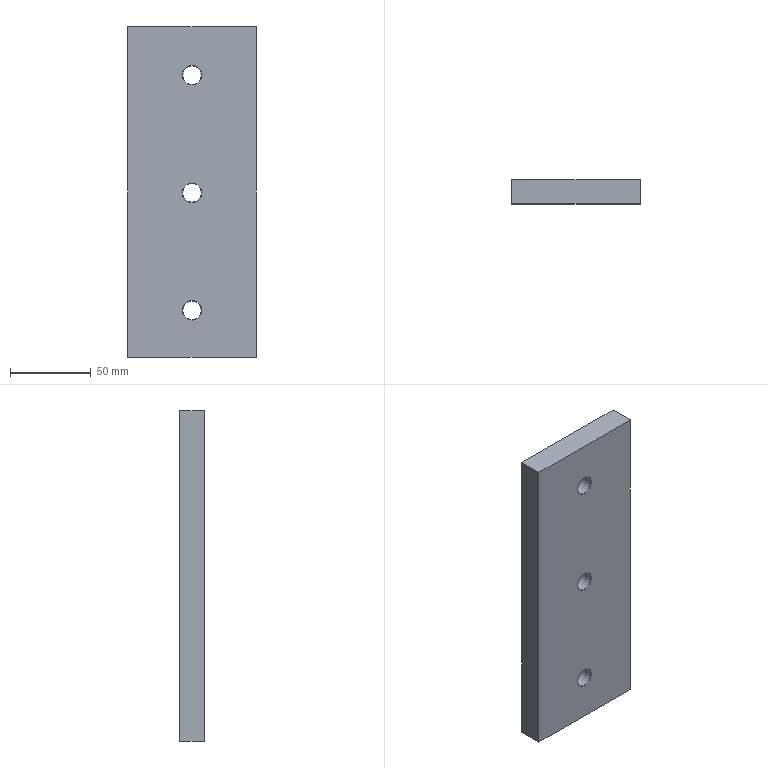Component | NX | CH3404_5-13_2 | 1 solid | 15 faces | box 80 x 15 x 205 mm | volume 241319 mm3 | plane 6 | cone 6 | cylinder 3 | commonest cylinder face diameters 11.5 x3
STEP:
#1=CARTESIAN_POINT('',(0.,0.,0.));
#2=DIRECTION('',(0.,0.,1.));
#3=DIRECTION('',(1.,0.,0.));
#4=AXIS2_PLACEMENT_3D('',#1,#2,#3);
#5=CARTESIAN_POINT('',(-275.,172.5,-10.));
#6=VERTEX_POINT('',#5);
#7=CARTESIAN_POINT('',(-275.,172.5,-215.));
#8=VERTEX_POINT('',#7);
#9=CARTESIAN_POINT('',(-275.,172.5,-10.));
#10=DIRECTION('',(0.,0.,-1.));
#11=VECTOR('',#10,1.);
#12=LINE('',#9,#11);
#13=CARTESIAN_POINT('',(-275.,187.5,-10.));
#14=DIRECTION('',(-1.,0.,0.));
#15=DIRECTION('',(0.,0.,1.));
#16=AXIS2_PLACEMENT_3D('',#13,#14,#15);
#17=PLANE('',#16);
#18=CARTESIAN_POINT('',(0.,-15.));
#19=DIRECTION('',(-1.,0.));
#20=VECTOR('',#19,1.);
#21=LINE('',#18,#20);
#22=(GEOMETRIC_REPRESENTATION_CONTEXT(2)PARAMETRIC_REPRESENTATION_CONTEXT()REPRESENTATION_CONTEXT('',''));
#23=DEFINITIONAL_REPRESENTATION('',(#21),#22);
#24=PCURVE('',#17,#23);
#25=CARTESIAN_POINT('',(-315.,172.5,-112.5));
#26=DIRECTION('',(0.,1.,0.));
#27=DIRECTION('',(0.,0.,-1.));
#28=AXIS2_PLACEMENT_3D('',#25,#26,#27);
#29=PLANE('',#28);
#30=CARTESIAN_POINT('',(-102.5,-40.));
#31=DIRECTION('',(1.,0.));
#32=VECTOR('',#31,1.);
#33=LINE('',#30,#32);
#34=(GEOMETRIC_REPRESENTATION_CONTEXT(2)PARAMETRIC_REPRESENTATION_CONTEXT()REPRESENTATION_CONTEXT('',''));
#35=DEFINITIONAL_REPRESENTATION('',(#33),#34);
#36=PCURVE('',#29,#35);
#37=SURFACE_CURVE('',#12,(#24,#36),.PCURVE_S1.);
#38=EDGE_CURVE('',#6,#8,#37,.T.);
#39=ORIENTED_EDGE('',*,*,#38,.T.);
#40=CARTESIAN_POINT('',(-275.,187.5,-215.));
#41=VERTEX_POINT('',#40);
#42=CARTESIAN_POINT('',(-275.,187.5,-215.));
#43=DIRECTION('',(0.,-1.,0.));
#44=VECTOR('',#43,1.);
#45=LINE('',#42,#44);
#46=CARTESIAN_POINT('',(-205.,0.));
#47=DIRECTION('',(0.,-1.));
#48=VECTOR('',#47,1.);
#49=LINE('',#46,#48);
#50=(GEOMETRIC_REPRESENTATION_CONTEXT(2)PARAMETRIC_REPRESENTATION_CONTEXT()REPRESENTATION_CONTEXT('',''));
#51=DEFINITIONAL_REPRESENTATION('',(#49),#50);
#52=PCURVE('',#17,#51);
#53=CARTESIAN_POINT('',(-275.,187.5,-215.));
#54=DIRECTION('',(0.,0.,1.));
#55=DIRECTION('',(0.,1.,0.));
#56=AXIS2_PLACEMENT_3D('',#53,#54,#55);
#57=PLANE('',#56);
#58=CARTESIAN_POINT('',(0.,0.));
#59=DIRECTION('',(-1.,0.));
#60=VECTOR('',#59,1.);
#61=LINE('',#58,#60);
#62=(GEOMETRIC_REPRESENTATION_CONTEXT(2)PARAMETRIC_REPRESENTATION_CONTEXT()REPRESENTATION_CONTEXT('',''));
#63=DEFINITIONAL_REPRESENTATION('',(#61),#62);
#64=PCURVE('',#57,#63);
#65=SURFACE_CURVE('',#45,(#52,#64),.PCURVE_S1.);
#66=EDGE_CURVE('',#41,#8,#65,.T.);
#67=ORIENTED_EDGE('',*,*,#66,.F.);
#68=CARTESIAN_POINT('',(-275.,187.5,-10.));
#69=VERTEX_POINT('',#68);
#70=CARTESIAN_POINT('',(-275.,187.5,-10.));
#71=DIRECTION('',(0.,0.,-1.));
#72=VECTOR('',#71,1.);
#73=LINE('',#70,#72);
#74=CARTESIAN_POINT('',(0.,0.));
#75=DIRECTION('',(-1.,0.));
#76=VECTOR('',#75,1.);
#77=LINE('',#74,#76);
#78=(GEOMETRIC_REPRESENTATION_CONTEXT(2)PARAMETRIC_REPRESENTATION_CONTEXT()REPRESENTATION_CONTEXT('',''));
#79=DEFINITIONAL_REPRESENTATION('',(#77),#78);
#80=PCURVE('',#17,#79);
#81=CARTESIAN_POINT('',(-315.,187.5,-112.5));
#82=DIRECTION('',(0.,1.,0.));
#83=DIRECTION('',(0.,0.,-1.));
#84=AXIS2_PLACEMENT_3D('',#81,#82,#83);
#85=PLANE('',#84);
#86=CARTESIAN_POINT('',(-102.5,-40.));
#87=DIRECTION('',(1.,0.));
#88=VECTOR('',#87,1.);
#89=LINE('',#86,#88);
#90=(GEOMETRIC_REPRESENTATION_CONTEXT(2)PARAMETRIC_REPRESENTATION_CONTEXT()REPRESENTATION_CONTEXT('',''));
#91=DEFINITIONAL_REPRESENTATION('',(#89),#90);
#92=PCURVE('',#85,#91);
#93=SURFACE_CURVE('',#73,(#80,#92),.PCURVE_S1.);
#94=EDGE_CURVE('',#69,#41,#93,.T.);
#95=ORIENTED_EDGE('',*,*,#94,.F.);
#96=CARTESIAN_POINT('',(-275.,187.5,-10.));
#97=DIRECTION('',(0.,-1.,0.));
#98=VECTOR('',#97,1.);
#99=LINE('',#96,#98);
#100=CARTESIAN_POINT('',(0.,0.));
#101=DIRECTION('',(0.,-1.));
#102=VECTOR('',#101,1.);
#103=LINE('',#100,#102);
#104=(GEOMETRIC_REPRESENTATION_CONTEXT(2)PARAMETRIC_REPRESENTATION_CONTEXT()REPRESENTATION_CONTEXT('',''));
#105=DEFINITIONAL_REPRESENTATION('',(#103),#104);
#106=PCURVE('',#17,#105);
#107=CARTESIAN_POINT('',(-355.,187.5,-10.));
#108=DIRECTION('',(0.,0.,-1.));
#109=DIRECTION('',(0.,-1.,0.));
#110=AXIS2_PLACEMENT_3D('',#107,#108,#109);
#111=PLANE('',#110);
#112=CARTESIAN_POINT('',(0.,-80.));
#113=DIRECTION('',(1.,0.));
#114=VECTOR('',#113,1.);
#115=LINE('',#112,#114);
#116=(GEOMETRIC_REPRESENTATION_CONTEXT(2)PARAMETRIC_REPRESENTATION_CONTEXT()REPRESENTATION_CONTEXT('',''));
#117=DEFINITIONAL_REPRESENTATION('',(#115),#116);
#118=PCURVE('',#111,#117);
#119=SURFACE_CURVE('',#99,(#106,#118),.PCURVE_S1.);
#120=EDGE_CURVE('',#69,#6,#119,.T.);
#121=ORIENTED_EDGE('',*,*,#120,.T.);
#122=EDGE_LOOP('',(#39,#67,#95,#121));
#123=FACE_BOUND('',#122,.T.);
#124=ADVANCED_FACE('',(#123),#17,.F.);
#125=CARTESIAN_POINT('',(-355.,172.5,-215.));
#126=VERTEX_POINT('',#125);
#127=CARTESIAN_POINT('',(-275.,172.5,-215.));
#128=DIRECTION('',(-1.,0.,0.));
#129=VECTOR('',#128,1.);
#130=LINE('',#127,#129);
#131=CARTESIAN_POINT('',(-15.,0.));
#132=DIRECTION('',(0.,1.));
#133=VECTOR('',#132,1.);
#134=LINE('',#131,#133);
#135=(GEOMETRIC_REPRESENTATION_CONTEXT(2)PARAMETRIC_REPRESENTATION_CONTEXT()REPRESENTATION_CONTEXT('',''));
#136=DEFINITIONAL_REPRESENTATION('',(#134),#135);
#137=PCURVE('',#57,#136);
#138=CARTESIAN_POINT('',(102.5,-40.));
#139=DIRECTION('',(0.,1.));
#140=VECTOR('',#139,1.);
#141=LINE('',#138,#140);
#142=(GEOMETRIC_REPRESENTATION_CONTEXT(2)PARAMETRIC_REPRESENTATION_CONTEXT()REPRESENTATION_CONTEXT('',''));
#143=DEFINITIONAL_REPRESENTATION('',(#141),#142);
#144=PCURVE('',#29,#143);
#145=SURFACE_CURVE('',#130,(#137,#144),.PCURVE_S1.);
#146=EDGE_CURVE('',#8,#126,#145,.T.);
#147=ORIENTED_EDGE('',*,*,#146,.T.);
#148=CARTESIAN_POINT('',(-355.,187.5,-215.));
#149=VERTEX_POINT('',#148);
#150=CARTESIAN_POINT('',(-355.,187.5,-215.));
#151=DIRECTION('',(0.,-1.,0.));
#152=VECTOR('',#151,1.);
#153=LINE('',#150,#152);
#154=CARTESIAN_POINT('',(0.,80.));
#155=DIRECTION('',(-1.,0.));
#156=VECTOR('',#155,1.);
#157=LINE('',#154,#156);
#158=(GEOMETRIC_REPRESENTATION_CONTEXT(2)PARAMETRIC_REPRESENTATION_CONTEXT()REPRESENTATION_CONTEXT('',''));
#159=DEFINITIONAL_REPRESENTATION('',(#157),#158);
#160=PCURVE('',#57,#159);
#161=CARTESIAN_POINT('',(-355.,187.5,-215.));
#162=DIRECTION('',(1.,0.,0.));
#163=DIRECTION('',(0.,0.,-1.));
#164=AXIS2_PLACEMENT_3D('',#161,#162,#163);
#165=PLANE('',#164);
#166=CARTESIAN_POINT('',(0.,0.));
#167=DIRECTION('',(0.,-1.));
#168=VECTOR('',#167,1.);
#169=LINE('',#166,#168);
#170=(GEOMETRIC_REPRESENTATION_CONTEXT(2)PARAMETRIC_REPRESENTATION_CONTEXT()REPRESENTATION_CONTEXT('',''));
#171=DEFINITIONAL_REPRESENTATION('',(#169),#170);
#172=PCURVE('',#165,#171);
#173=SURFACE_CURVE('',#153,(#160,#172),.PCURVE_S1.);
#174=EDGE_CURVE('',#149,#126,#173,.T.);
#175=ORIENTED_EDGE('',*,*,#174,.F.);
#176=CARTESIAN_POINT('',(-275.,187.5,-215.));
#177=DIRECTION('',(-1.,0.,0.));
#178=VECTOR('',#177,1.);
#179=LINE('',#176,#178);
#180=CARTESIAN_POINT('',(0.,0.));
#181=DIRECTION('',(0.,1.));
#182=VECTOR('',#181,1.);
#183=LINE('',#180,#182);
#184=(GEOMETRIC_REPRESENTATION_CONTEXT(2)PARAMETRIC_REPRESENTATION_CONTEXT()REPRESENTATION_CONTEXT('',''));
#185=DEFINITIONAL_REPRESENTATION('',(#183),#184);
#186=PCURVE('',#57,#185);
#187=CARTESIAN_POINT('',(102.5,-40.));
#188=DIRECTION('',(0.,1.));
#189=VECTOR('',#188,1.);
#190=LINE('',#187,#189);
#191=(GEOMETRIC_REPRESENTATION_CONTEXT(2)PARAMETRIC_REPRESENTATION_CONTEXT()REPRESENTATION_CONTEXT('',''));
#192=DEFINITIONAL_REPRESENTATION('',(#190),#191);
#193=PCURVE('',#85,#192);
#194=SURFACE_CURVE('',#179,(#186,#193),.PCURVE_S1.);
#195=EDGE_CURVE('',#41,#149,#194,.T.);
#196=ORIENTED_EDGE('',*,*,#195,.F.);
#197=ORIENTED_EDGE('',*,*,#66,.T.);
#198=EDGE_LOOP('',(#147,#175,#196,#197));
#199=FACE_BOUND('',#198,.T.);
#200=ADVANCED_FACE('',(#199),#57,.F.);
#201=CARTESIAN_POINT('',(-355.,172.5,-10.));
#202=VERTEX_POINT('',#201);
#203=CARTESIAN_POINT('',(-355.,172.5,-215.));
#204=DIRECTION('',(0.,0.,1.));
#205=VECTOR('',#204,1.);
#206=LINE('',#203,#205);
#207=CARTESIAN_POINT('',(0.,-15.));
#208=DIRECTION('',(-1.,0.));
#209=VECTOR('',#208,1.);
#210=LINE('',#207,#209);
#211=(GEOMETRIC_REPRESENTATION_CONTEXT(2)PARAMETRIC_REPRESENTATION_CONTEXT()REPRESENTATION_CONTEXT('',''));
#212=DEFINITIONAL_REPRESENTATION('',(#210),#211);
#213=PCURVE('',#165,#212);
#214=CARTESIAN_POINT('',(102.5,40.));
#215=DIRECTION('',(-1.,0.));
#216=VECTOR('',#215,1.);
#217=LINE('',#214,#216);
#218=(GEOMETRIC_REPRESENTATION_CONTEXT(2)PARAMETRIC_REPRESENTATION_CONTEXT()REPRESENTATION_CONTEXT('',''));
#219=DEFINITIONAL_REPRESENTATION('',(#217),#218);
#220=PCURVE('',#29,#219);
#221=SURFACE_CURVE('',#206,(#213,#220),.PCURVE_S1.);
#222=EDGE_CURVE('',#126,#202,#221,.T.);
#223=ORIENTED_EDGE('',*,*,#222,.T.);
#224=CARTESIAN_POINT('',(-355.,187.5,-10.));
#225=VERTEX_POINT('',#224);
#226=CARTESIAN_POINT('',(-355.,187.5,-10.));
#227=DIRECTION('',(0.,-1.,0.));
#228=VECTOR('',#227,1.);
#229=LINE('',#226,#228);
#230=CARTESIAN_POINT('',(-205.,0.));
#231=DIRECTION('',(0.,-1.));
#232=VECTOR('',#231,1.);
#233=LINE('',#230,#232);
#234=(GEOMETRIC_REPRESENTATION_CONTEXT(2)PARAMETRIC_REPRESENTATION_CONTEXT()REPRESENTATION_CONTEXT('',''));
#235=DEFINITIONAL_REPRESENTATION('',(#233),#234);
#236=PCURVE('',#165,#235);
#237=CARTESIAN_POINT('',(0.,0.));
#238=DIRECTION('',(1.,0.));
#239=VECTOR('',#238,1.);
#240=LINE('',#237,#239);
#241=(GEOMETRIC_REPRESENTATION_CONTEXT(2)PARAMETRIC_REPRESENTATION_CONTEXT()REPRESENTATION_CONTEXT('',''));
#242=DEFINITIONAL_REPRESENTATION('',(#240),#241);
#243=PCURVE('',#111,#242);
#244=SURFACE_CURVE('',#229,(#236,#243),.PCURVE_S1.);
#245=EDGE_CURVE('',#225,#202,#244,.T.);
#246=ORIENTED_EDGE('',*,*,#245,.F.);
#247=CARTESIAN_POINT('',(-355.,187.5,-215.));
#248=DIRECTION('',(0.,0.,1.));
#249=VECTOR('',#248,1.);
#250=LINE('',#247,#249);
#251=CARTESIAN_POINT('',(0.,0.));
#252=DIRECTION('',(-1.,0.));
#253=VECTOR('',#252,1.);
#254=LINE('',#251,#253);
#255=(GEOMETRIC_REPRESENTATION_CONTEXT(2)PARAMETRIC_REPRESENTATION_CONTEXT()REPRESENTATION_CONTEXT('',''));
#256=DEFINITIONAL_REPRESENTATION('',(#254),#255);
#257=PCURVE('',#165,#256);
#258=CARTESIAN_POINT('',(102.5,40.));
#259=DIRECTION('',(-1.,0.));
#260=VECTOR('',#259,1.);
#261=LINE('',#258,#260);
#262=(GEOMETRIC_REPRESENTATION_CONTEXT(2)PARAMETRIC_REPRESENTATION_CONTEXT()REPRESENTATION_CONTEXT('',''));
#263=DEFINITIONAL_REPRESENTATION('',(#261),#262);
#264=PCURVE('',#85,#263);
#265=SURFACE_CURVE('',#250,(#257,#264),.PCURVE_S1.);
#266=EDGE_CURVE('',#149,#225,#265,.T.);
#267=ORIENTED_EDGE('',*,*,#266,.F.);
#268=ORIENTED_EDGE('',*,*,#174,.T.);
#269=EDGE_LOOP('',(#223,#246,#267,#268));
#270=FACE_BOUND('',#269,.T.);
#271=ADVANCED_FACE('',(#270),#165,.F.);
#272=CARTESIAN_POINT('',(-355.,172.5,-10.));
#273=DIRECTION('',(1.,0.,0.));
#274=VECTOR('',#273,1.);
#275=LINE('',#272,#274);
#276=CARTESIAN_POINT('',(15.,0.));
#277=DIRECTION('',(0.,-1.));
#278=VECTOR('',#277,1.);
#279=LINE('',#276,#278);
#280=(GEOMETRIC_REPRESENTATION_CONTEXT(2)PARAMETRIC_REPRESENTATION_CONTEXT()REPRESENTATION_CONTEXT('',''));
#281=DEFINITIONAL_REPRESENTATION('',(#279),#280);
#282=PCURVE('',#111,#281);
#283=CARTESIAN_POINT('',(-102.5,40.));
#284=DIRECTION('',(0.,-1.));
#285=VECTOR('',#284,1.);
#286=LINE('',#283,#285);
#287=(GEOMETRIC_REPRESENTATION_CONTEXT(2)PARAMETRIC_REPRESENTATION_CONTEXT()REPRESENTATION_CONTEXT('',''));
#288=DEFINITIONAL_REPRESENTATION('',(#286),#287);
#289=PCURVE('',#29,#288);
#290=SURFACE_CURVE('',#275,(#282,#289),.PCURVE_S1.);
#291=EDGE_CURVE('',#202,#6,#290,.T.);
#292=ORIENTED_EDGE('',*,*,#291,.T.);
#293=ORIENTED_EDGE('',*,*,#120,.F.);
#294=CARTESIAN_POINT('',(-355.,187.5,-10.));
#295=DIRECTION('',(1.,0.,0.));
#296=VECTOR('',#295,1.);
#297=LINE('',#294,#296);
#298=CARTESIAN_POINT('',(0.,0.));
#299=DIRECTION('',(0.,-1.));
#300=VECTOR('',#299,1.);
#301=LINE('',#298,#300);
#302=(GEOMETRIC_REPRESENTATION_CONTEXT(2)PARAMETRIC_REPRESENTATION_CONTEXT()REPRESENTATION_CONTEXT('',''));
#303=DEFINITIONAL_REPRESENTATION('',(#301),#302);
#304=PCURVE('',#111,#303);
#305=CARTESIAN_POINT('',(-102.5,40.));
#306=DIRECTION('',(0.,-1.));
#307=VECTOR('',#306,1.);
#308=LINE('',#305,#307);
#309=(GEOMETRIC_REPRESENTATION_CONTEXT(2)PARAMETRIC_REPRESENTATION_CONTEXT()REPRESENTATION_CONTEXT('',''));
#310=DEFINITIONAL_REPRESENTATION('',(#308),#309);
#311=PCURVE('',#85,#310);
#312=SURFACE_CURVE('',#297,(#304,#311),.PCURVE_S1.);
#313=EDGE_CURVE('',#225,#69,#312,.T.);
#314=ORIENTED_EDGE('',*,*,#313,.F.);
#315=ORIENTED_EDGE('',*,*,#245,.T.);
#316=EDGE_LOOP('',(#292,#293,#314,#315));
#317=FACE_BOUND('',#316,.T.);
#318=ADVANCED_FACE('',(#317),#111,.F.);
#319=CARTESIAN_POINT('',(-315.,187.5,-46.));
#320=VERTEX_POINT('',#319);
#321=CARTESIAN_POINT('',(-315.,187.5,-40.));
#322=DIRECTION('',(0.,-1.,0.));
#323=DIRECTION('',(0.,0.,-1.));
#324=AXIS2_PLACEMENT_3D('',#321,#322,#323);
#325=CIRCLE('',#324,6.);
#326=CARTESIAN_POINT('',(-66.5,0.));
#327=CARTESIAN_POINT('',(-66.5,-10.392));
#328=CARTESIAN_POINT('',(-75.5,-5.196));
#329=CARTESIAN_POINT('',(-84.5,-0.));
#330=CARTESIAN_POINT('',(-75.5,5.196));
#331=CARTESIAN_POINT('',(-66.5,10.392));
#332=CARTESIAN_POINT('',(-66.5,0.));
#333=(BOUNDED_CURVE()B_SPLINE_CURVE(2,(#326,#327,#328,#329,#330,#331,#332),.UNSPECIFIED.,.T.,.F.)B_SPLINE_CURVE_WITH_KNOTS((1,2,2,2,2,1),(-2.094,0.,2.094,4.189,6.283,8.378),.UNSPECIFIED.)CURVE()GEOMETRIC_REPRESENTATION_ITEM()RATIONAL_B_SPLINE_CURVE((1.,0.5,1.,0.5,1.,0.5,1.))REPRESENTATION_ITEM(''));
#334=(GEOMETRIC_REPRESENTATION_CONTEXT(2)PARAMETRIC_REPRESENTATION_CONTEXT()REPRESENTATION_CONTEXT('',''));
#335=DEFINITIONAL_REPRESENTATION('',(#333),#334);
#336=PCURVE('',#85,#335);
#337=CARTESIAN_POINT('',(-315.,187.5,-40.));
#338=DIRECTION('',(0.,1.,0.));
#339=DIRECTION('',(0.,0.,-1.));
#340=AXIS2_PLACEMENT_3D('',#337,#338,#339);
#341=CONICAL_SURFACE('',#340,6.,0.7854);
#342=CARTESIAN_POINT('',(6.283,-0.));
#343=DIRECTION('',(-1.,0.));
#344=VECTOR('',#343,1.);
#345=LINE('',#342,#344);
#346=(GEOMETRIC_REPRESENTATION_CONTEXT(2)PARAMETRIC_REPRESENTATION_CONTEXT()REPRESENTATION_CONTEXT('',''));
#347=DEFINITIONAL_REPRESENTATION('',(#345),#346);
#348=PCURVE('',#341,#347);
#349=SURFACE_CURVE('',#325,(#336,#348),.PCURVE_S1.);
#350=EDGE_CURVE('',#320,#320,#349,.T.);
#351=ORIENTED_EDGE('',*,*,#350,.T.);
#352=EDGE_LOOP('',(#351));
#353=FACE_BOUND('',#352,.T.);
#354=CARTESIAN_POINT('',(-315.,187.5,-119.));
#355=VERTEX_POINT('',#354);
#356=CARTESIAN_POINT('',(-315.,187.5,-113.));
#357=DIRECTION('',(0.,-1.,0.));
#358=DIRECTION('',(0.,0.,-1.));
#359=AXIS2_PLACEMENT_3D('',#356,#357,#358);
#360=CIRCLE('',#359,6.);
#361=CARTESIAN_POINT('',(6.5,0.));
#362=CARTESIAN_POINT('',(6.5,-10.392));
#363=CARTESIAN_POINT('',(-2.5,-5.196));
#364=CARTESIAN_POINT('',(-11.5,-0.));
#365=CARTESIAN_POINT('',(-2.5,5.196));
#366=CARTESIAN_POINT('',(6.5,10.392));
#367=CARTESIAN_POINT('',(6.5,0.));
#368=(BOUNDED_CURVE()B_SPLINE_CURVE(2,(#361,#362,#363,#364,#365,#366,#367),.UNSPECIFIED.,.T.,.F.)B_SPLINE_CURVE_WITH_KNOTS((1,2,2,2,2,1),(-2.094,0.,2.094,4.189,6.283,8.378),.UNSPECIFIED.)CURVE()GEOMETRIC_REPRESENTATION_ITEM()RATIONAL_B_SPLINE_CURVE((1.,0.5,1.,0.5,1.,0.5,1.))REPRESENTATION_ITEM(''));
#369=(GEOMETRIC_REPRESENTATION_CONTEXT(2)PARAMETRIC_REPRESENTATION_CONTEXT()REPRESENTATION_CONTEXT('',''));
#370=DEFINITIONAL_REPRESENTATION('',(#368),#369);
#371=PCURVE('',#85,#370);
#372=CARTESIAN_POINT('',(-315.,187.5,-113.));
#373=DIRECTION('',(0.,1.,0.));
#374=DIRECTION('',(0.,0.,-1.));
#375=AXIS2_PLACEMENT_3D('',#372,#373,#374);
#376=CONICAL_SURFACE('',#375,6.,0.7854);
#377=CARTESIAN_POINT('',(6.283,0.));
#378=DIRECTION('',(-1.,0.));
#379=VECTOR('',#378,1.);
#380=LINE('',#377,#379);
#381=(GEOMETRIC_REPRESENTATION_CONTEXT(2)PARAMETRIC_REPRESENTATION_CONTEXT()REPRESENTATION_CONTEXT('',''));
#382=DEFINITIONAL_REPRESENTATION('',(#380),#381);
#383=PCURVE('',#376,#382);
#384=SURFACE_CURVE('',#360,(#371,#383),.PCURVE_S1.);
#385=EDGE_CURVE('',#355,#355,#384,.T.);
#386=ORIENTED_EDGE('',*,*,#385,.T.);
#387=EDGE_LOOP('',(#386));
#388=FACE_BOUND('',#387,.T.);
#389=CARTESIAN_POINT('',(-315.,187.5,-192.));
#390=VERTEX_POINT('',#389);
#391=CARTESIAN_POINT('',(-315.,187.5,-186.));
#392=DIRECTION('',(0.,-1.,0.));
#393=DIRECTION('',(0.,0.,-1.));
#394=AXIS2_PLACEMENT_3D('',#391,#392,#393);
#395=CIRCLE('',#394,6.);
#396=CARTESIAN_POINT('',(79.5,0.));
#397=CARTESIAN_POINT('',(79.5,-10.392));
#398=CARTESIAN_POINT('',(70.5,-5.196));
#399=CARTESIAN_POINT('',(61.5,-0.));
#400=CARTESIAN_POINT('',(70.5,5.196));
#401=CARTESIAN_POINT('',(79.5,10.392));
#402=CARTESIAN_POINT('',(79.5,0.));
#403=(BOUNDED_CURVE()B_SPLINE_CURVE(2,(#396,#397,#398,#399,#400,#401,#402),.UNSPECIFIED.,.T.,.F.)B_SPLINE_CURVE_WITH_KNOTS((1,2,2,2,2,1),(-2.094,0.,2.094,4.189,6.283,8.378),.UNSPECIFIED.)CURVE()GEOMETRIC_REPRESENTATION_ITEM()RATIONAL_B_SPLINE_CURVE((1.,0.5,1.,0.5,1.,0.5,1.))REPRESENTATION_ITEM(''));
#404=(GEOMETRIC_REPRESENTATION_CONTEXT(2)PARAMETRIC_REPRESENTATION_CONTEXT()REPRESENTATION_CONTEXT('',''));
#405=DEFINITIONAL_REPRESENTATION('',(#403),#404);
#406=PCURVE('',#85,#405);
#407=CARTESIAN_POINT('',(-315.,187.5,-186.));
#408=DIRECTION('',(0.,1.,0.));
#409=DIRECTION('',(0.,0.,-1.));
#410=AXIS2_PLACEMENT_3D('',#407,#408,#409);
#411=CONICAL_SURFACE('',#410,6.,0.7854);
#412=CARTESIAN_POINT('',(6.283,-0.));
#413=DIRECTION('',(-1.,0.));
#414=VECTOR('',#413,1.);
#415=LINE('',#412,#414);
#416=(GEOMETRIC_REPRESENTATION_CONTEXT(2)PARAMETRIC_REPRESENTATION_CONTEXT()REPRESENTATION_CONTEXT('',''));
#417=DEFINITIONAL_REPRESENTATION('',(#415),#416);
#418=PCURVE('',#411,#417);
#419=SURFACE_CURVE('',#395,(#406,#418),.PCURVE_S1.);
#420=EDGE_CURVE('',#390,#390,#419,.T.);
#421=ORIENTED_EDGE('',*,*,#420,.T.);
#422=EDGE_LOOP('',(#421));
#423=FACE_BOUND('',#422,.T.);
#424=ORIENTED_EDGE('',*,*,#94,.T.);
#425=ORIENTED_EDGE('',*,*,#195,.T.);
#426=ORIENTED_EDGE('',*,*,#266,.T.);
#427=ORIENTED_EDGE('',*,*,#313,.T.);
#428=EDGE_LOOP('',(#424,#425,#426,#427));
#429=FACE_BOUND('',#428,.T.);
#430=ADVANCED_FACE('',(#353,#388,#423,#429),#85,.T.);
#431=CARTESIAN_POINT('',(-315.,172.5,-46.));
#432=VERTEX_POINT('',#431);
#433=CARTESIAN_POINT('',(-315.,172.5,-40.));
#434=DIRECTION('',(0.,1.,0.));
#435=DIRECTION('',(0.,0.,-1.));
#436=AXIS2_PLACEMENT_3D('',#433,#434,#435);
#437=CIRCLE('',#436,6.);
#438=CARTESIAN_POINT('',(-72.5,0.));
#439=DIRECTION('',(1.,0.));
#440=AXIS2_PLACEMENT_2D('',#438,#439);
#441=CIRCLE('',#440,6.);
#442=(GEOMETRIC_REPRESENTATION_CONTEXT(2)PARAMETRIC_REPRESENTATION_CONTEXT()REPRESENTATION_CONTEXT('',''));
#443=DEFINITIONAL_REPRESENTATION('',(#441),#442);
#444=PCURVE('',#29,#443);
#445=CARTESIAN_POINT('',(-315.,172.5,-40.));
#446=DIRECTION('',(0.,-1.,0.));
#447=DIRECTION('',(0.,0.,1.));
#448=AXIS2_PLACEMENT_3D('',#445,#446,#447);
#449=CONICAL_SURFACE('',#448,6.,0.7854);
#450=CARTESIAN_POINT('',(9.425,-0.));
#451=DIRECTION('',(-1.,0.));
#452=VECTOR('',#451,1.);
#453=LINE('',#450,#452);
#454=(GEOMETRIC_REPRESENTATION_CONTEXT(2)PARAMETRIC_REPRESENTATION_CONTEXT()REPRESENTATION_CONTEXT('',''));
#455=DEFINITIONAL_REPRESENTATION('',(#453),#454);
#456=PCURVE('',#449,#455);
#457=SURFACE_CURVE('',#437,(#444,#456),.PCURVE_S1.);
#458=EDGE_CURVE('',#432,#432,#457,.T.);
#459=ORIENTED_EDGE('',*,*,#458,.T.);
#460=EDGE_LOOP('',(#459));
#461=FACE_BOUND('',#460,.T.);
#462=CARTESIAN_POINT('',(-315.,172.5,-119.));
#463=VERTEX_POINT('',#462);
#464=CARTESIAN_POINT('',(-315.,172.5,-113.));
#465=DIRECTION('',(0.,1.,0.));
#466=DIRECTION('',(0.,0.,-1.));
#467=AXIS2_PLACEMENT_3D('',#464,#465,#466);
#468=CIRCLE('',#467,6.);
#469=CARTESIAN_POINT('',(0.5,0.));
#470=DIRECTION('',(1.,0.));
#471=AXIS2_PLACEMENT_2D('',#469,#470);
#472=CIRCLE('',#471,6.);
#473=(GEOMETRIC_REPRESENTATION_CONTEXT(2)PARAMETRIC_REPRESENTATION_CONTEXT()REPRESENTATION_CONTEXT('',''));
#474=DEFINITIONAL_REPRESENTATION('',(#472),#473);
#475=PCURVE('',#29,#474);
#476=CARTESIAN_POINT('',(-315.,172.5,-113.));
#477=DIRECTION('',(0.,-1.,0.));
#478=DIRECTION('',(0.,0.,1.));
#479=AXIS2_PLACEMENT_3D('',#476,#477,#478);
#480=CONICAL_SURFACE('',#479,6.,0.7854);
#481=CARTESIAN_POINT('',(9.425,0.));
#482=DIRECTION('',(-1.,0.));
#483=VECTOR('',#482,1.);
#484=LINE('',#481,#483);
#485=(GEOMETRIC_REPRESENTATION_CONTEXT(2)PARAMETRIC_REPRESENTATION_CONTEXT()REPRESENTATION_CONTEXT('',''));
#486=DEFINITIONAL_REPRESENTATION('',(#484),#485);
#487=PCURVE('',#480,#486);
#488=SURFACE_CURVE('',#468,(#475,#487),.PCURVE_S1.);
#489=EDGE_CURVE('',#463,#463,#488,.T.);
#490=ORIENTED_EDGE('',*,*,#489,.T.);
#491=EDGE_LOOP('',(#490));
#492=FACE_BOUND('',#491,.T.);
#493=CARTESIAN_POINT('',(-315.,172.5,-192.));
#494=VERTEX_POINT('',#493);
#495=CARTESIAN_POINT('',(-315.,172.5,-186.));
#496=DIRECTION('',(0.,1.,0.));
#497=DIRECTION('',(0.,0.,-1.));
#498=AXIS2_PLACEMENT_3D('',#495,#496,#497);
#499=CIRCLE('',#498,6.);
#500=CARTESIAN_POINT('',(73.5,0.));
#501=DIRECTION('',(1.,0.));
#502=AXIS2_PLACEMENT_2D('',#500,#501);
#503=CIRCLE('',#502,6.);
#504=(GEOMETRIC_REPRESENTATION_CONTEXT(2)PARAMETRIC_REPRESENTATION_CONTEXT()REPRESENTATION_CONTEXT('',''));
#505=DEFINITIONAL_REPRESENTATION('',(#503),#504);
#506=PCURVE('',#29,#505);
#507=CARTESIAN_POINT('',(-315.,172.5,-186.));
#508=DIRECTION('',(0.,-1.,0.));
#509=DIRECTION('',(0.,0.,1.));
#510=AXIS2_PLACEMENT_3D('',#507,#508,#509);
#511=CONICAL_SURFACE('',#510,6.,0.7854);
#512=CARTESIAN_POINT('',(9.425,-0.));
#513=DIRECTION('',(-1.,0.));
#514=VECTOR('',#513,1.);
#515=LINE('',#512,#514);
#516=(GEOMETRIC_REPRESENTATION_CONTEXT(2)PARAMETRIC_REPRESENTATION_CONTEXT()REPRESENTATION_CONTEXT('',''));
#517=DEFINITIONAL_REPRESENTATION('',(#515),#516);
#518=PCURVE('',#511,#517);
#519=SURFACE_CURVE('',#499,(#506,#518),.PCURVE_S1.);
#520=EDGE_CURVE('',#494,#494,#519,.T.);
#521=ORIENTED_EDGE('',*,*,#520,.T.);
#522=EDGE_LOOP('',(#521));
#523=FACE_BOUND('',#522,.T.);
#524=ORIENTED_EDGE('',*,*,#38,.F.);
#525=ORIENTED_EDGE('',*,*,#291,.F.);
#526=ORIENTED_EDGE('',*,*,#222,.F.);
#527=ORIENTED_EDGE('',*,*,#146,.F.);
#528=EDGE_LOOP('',(#524,#525,#526,#527));
#529=FACE_BOUND('',#528,.T.);
#530=ADVANCED_FACE('',(#461,#492,#523,#529),#29,.F.);
#531=CARTESIAN_POINT('',(-315.,172.75,-191.75));
#532=VERTEX_POINT('',#531);
#533=CARTESIAN_POINT('',(-315.,172.75,-186.));
#534=DIRECTION('',(0.,-1.,0.));
#535=DIRECTION('',(0.,0.,-1.));
#536=AXIS2_PLACEMENT_3D('',#533,#534,#535);
#537=CIRCLE('',#536,5.75);
#538=CARTESIAN_POINT('',(-315.,187.5,-186.));
#539=DIRECTION('',(0.,-1.,0.));
#540=DIRECTION('',(0.,0.,1.));
#541=AXIS2_PLACEMENT_3D('',#538,#539,#540);
#542=CYLINDRICAL_SURFACE('',#541,5.75);
#543=CARTESIAN_POINT('',(3.142,14.75));
#544=DIRECTION('',(1.,0.));
#545=VECTOR('',#544,1.);
#546=LINE('',#543,#545);
#547=(GEOMETRIC_REPRESENTATION_CONTEXT(2)PARAMETRIC_REPRESENTATION_CONTEXT()REPRESENTATION_CONTEXT('',''));
#548=DEFINITIONAL_REPRESENTATION('',(#546),#547);
#549=PCURVE('',#542,#548);
#550=CARTESIAN_POINT('',(3.142,-0.25));
#551=DIRECTION('',(1.,0.));
#552=VECTOR('',#551,1.);
#553=LINE('',#550,#552);
#554=(GEOMETRIC_REPRESENTATION_CONTEXT(2)PARAMETRIC_REPRESENTATION_CONTEXT()REPRESENTATION_CONTEXT('',''));
#555=DEFINITIONAL_REPRESENTATION('',(#553),#554);
#556=PCURVE('',#511,#555);
#557=SURFACE_CURVE('',#537,(#549,#556),.PCURVE_S1.);
#558=EDGE_CURVE('',#532,#532,#557,.T.);
#559=ORIENTED_EDGE('',*,*,#558,.F.);
#560=CARTESIAN_POINT('',(-315.,187.25,-191.75));
#561=VERTEX_POINT('',#560);
#562=CARTESIAN_POINT('',(-315.,187.25,-191.75));
#563=CARTESIAN_POINT('',(-315.,172.75,-191.75));
#564=B_SPLINE_CURVE_WITH_KNOTS('',1,(#562,#563),.UNSPECIFIED.,.F.,.F.,(2,2),(0.25,14.75),.PIECEWISE_BEZIER_KNOTS.);
#565=CARTESIAN_POINT('',(3.142,0.));
#566=DIRECTION('',(0.,1.));
#567=VECTOR('',#566,1.);
#568=LINE('',#565,#567);
#569=(GEOMETRIC_REPRESENTATION_CONTEXT(2)PARAMETRIC_REPRESENTATION_CONTEXT()REPRESENTATION_CONTEXT('',''));
#570=DEFINITIONAL_REPRESENTATION('',(#568),#569);
#571=PCURVE('',#542,#570);
#572=CARTESIAN_POINT('',(9.425,0.));
#573=DIRECTION('',(0.,1.));
#574=VECTOR('',#573,1.);
#575=LINE('',#572,#574);
#576=(GEOMETRIC_REPRESENTATION_CONTEXT(2)PARAMETRIC_REPRESENTATION_CONTEXT()REPRESENTATION_CONTEXT('',''));
#577=DEFINITIONAL_REPRESENTATION('',(#575),#576);
#578=PCURVE('',#542,#577);
#579=SEAM_CURVE('',#564,(#571,#578),.PCURVE_S1.);
#580=EDGE_CURVE('',#561,#532,#579,.T.);
#581=ORIENTED_EDGE('',*,*,#580,.F.);
#582=CARTESIAN_POINT('',(-315.,187.25,-186.));
#583=DIRECTION('',(0.,1.,0.));
#584=DIRECTION('',(0.,0.,-1.));
#585=AXIS2_PLACEMENT_3D('',#582,#583,#584);
#586=CIRCLE('',#585,5.75);
#587=CARTESIAN_POINT('',(9.425,0.25));
#588=DIRECTION('',(-1.,0.));
#589=VECTOR('',#588,1.);
#590=LINE('',#587,#589);
#591=(GEOMETRIC_REPRESENTATION_CONTEXT(2)PARAMETRIC_REPRESENTATION_CONTEXT()REPRESENTATION_CONTEXT('',''));
#592=DEFINITIONAL_REPRESENTATION('',(#590),#591);
#593=PCURVE('',#542,#592);
#594=CARTESIAN_POINT('',(0.,-0.25));
#595=DIRECTION('',(1.,0.));
#596=VECTOR('',#595,1.);
#597=LINE('',#594,#596);
#598=(GEOMETRIC_REPRESENTATION_CONTEXT(2)PARAMETRIC_REPRESENTATION_CONTEXT()REPRESENTATION_CONTEXT('',''));
#599=DEFINITIONAL_REPRESENTATION('',(#597),#598);
#600=PCURVE('',#411,#599);
#601=SURFACE_CURVE('',#586,(#593,#600),.PCURVE_S1.);
#602=EDGE_CURVE('',#561,#561,#601,.T.);
#603=ORIENTED_EDGE('',*,*,#602,.F.);
#604=ORIENTED_EDGE('',*,*,#580,.T.);
#605=EDGE_LOOP('',(#559,#581,#603,#604));
#606=FACE_BOUND('',#605,.F.);
#607=ADVANCED_FACE('',(#606),#542,.F.);
#608=ORIENTED_EDGE('',*,*,#602,.T.);
#609=CARTESIAN_POINT('',(-315.,187.25,-191.75));
#610=CARTESIAN_POINT('',(-315.,187.5,-192.));
#611=B_SPLINE_CURVE_WITH_KNOTS('',1,(#609,#610),.UNSPECIFIED.,.F.,.F.,(2,2),(-0.3536,-0.),.PIECEWISE_BEZIER_KNOTS.);
#612=CARTESIAN_POINT('',(6.283,0.));
#613=DIRECTION('',(0.,1.));
#614=VECTOR('',#613,1.);
#615=LINE('',#612,#614);
#616=(GEOMETRIC_REPRESENTATION_CONTEXT(2)PARAMETRIC_REPRESENTATION_CONTEXT()REPRESENTATION_CONTEXT('',''));
#617=DEFINITIONAL_REPRESENTATION('',(#615),#616);
#618=PCURVE('',#411,#617);
#619=CARTESIAN_POINT('',(0.,0.));
#620=DIRECTION('',(0.,1.));
#621=VECTOR('',#620,1.);
#622=LINE('',#619,#621);
#623=(GEOMETRIC_REPRESENTATION_CONTEXT(2)PARAMETRIC_REPRESENTATION_CONTEXT()REPRESENTATION_CONTEXT('',''));
#624=DEFINITIONAL_REPRESENTATION('',(#622),#623);
#625=PCURVE('',#411,#624);
#626=SEAM_CURVE('',#611,(#618,#625),.PCURVE_S1.);
#627=EDGE_CURVE('',#561,#390,#626,.T.);
#628=ORIENTED_EDGE('',*,*,#627,.T.);
#629=ORIENTED_EDGE('',*,*,#420,.T.);
#630=ORIENTED_EDGE('',*,*,#627,.F.);
#631=EDGE_LOOP('',(#608,#628,#629,#630));
#632=FACE_BOUND('',#631,.F.);
#633=ADVANCED_FACE('',(#632),#411,.F.);
#634=ORIENTED_EDGE('',*,*,#558,.T.);
#635=CARTESIAN_POINT('',(-315.,172.75,-191.75));
#636=CARTESIAN_POINT('',(-315.,172.5,-192.));
#637=B_SPLINE_CURVE_WITH_KNOTS('',1,(#635,#636),.UNSPECIFIED.,.F.,.F.,(2,2),(-0.3536,-0.),.PIECEWISE_BEZIER_KNOTS.);
#638=CARTESIAN_POINT('',(9.425,0.));
#639=DIRECTION('',(0.,1.));
#640=VECTOR('',#639,1.);
#641=LINE('',#638,#640);
#642=(GEOMETRIC_REPRESENTATION_CONTEXT(2)PARAMETRIC_REPRESENTATION_CONTEXT()REPRESENTATION_CONTEXT('',''));
#643=DEFINITIONAL_REPRESENTATION('',(#641),#642);
#644=PCURVE('',#511,#643);
#645=CARTESIAN_POINT('',(3.142,0.));
#646=DIRECTION('',(0.,1.));
#647=VECTOR('',#646,1.);
#648=LINE('',#645,#647);
#649=(GEOMETRIC_REPRESENTATION_CONTEXT(2)PARAMETRIC_REPRESENTATION_CONTEXT()REPRESENTATION_CONTEXT('',''));
#650=DEFINITIONAL_REPRESENTATION('',(#648),#649);
#651=PCURVE('',#511,#650);
#652=SEAM_CURVE('',#637,(#644,#651),.PCURVE_S1.);
#653=EDGE_CURVE('',#532,#494,#652,.T.);
#654=ORIENTED_EDGE('',*,*,#653,.T.);
#655=ORIENTED_EDGE('',*,*,#520,.T.);
#656=ORIENTED_EDGE('',*,*,#653,.F.);
#657=EDGE_LOOP('',(#634,#654,#655,#656));
#658=FACE_BOUND('',#657,.F.);
#659=ADVANCED_FACE('',(#658),#511,.F.);
#660=CARTESIAN_POINT('',(-315.,172.75,-118.75));
#661=VERTEX_POINT('',#660);
#662=CARTESIAN_POINT('',(-315.,172.75,-113.));
#663=DIRECTION('',(0.,-1.,0.));
#664=DIRECTION('',(0.,0.,-1.));
#665=AXIS2_PLACEMENT_3D('',#662,#663,#664);
#666=CIRCLE('',#665,5.75);
#667=CARTESIAN_POINT('',(-315.,187.5,-113.));
#668=DIRECTION('',(0.,-1.,0.));
#669=DIRECTION('',(0.,0.,1.));
#670=AXIS2_PLACEMENT_3D('',#667,#668,#669);
#671=CYLINDRICAL_SURFACE('',#670,5.75);
#672=CARTESIAN_POINT('',(3.142,14.75));
#673=DIRECTION('',(1.,0.));
#674=VECTOR('',#673,1.);
#675=LINE('',#672,#674);
#676=(GEOMETRIC_REPRESENTATION_CONTEXT(2)PARAMETRIC_REPRESENTATION_CONTEXT()REPRESENTATION_CONTEXT('',''));
#677=DEFINITIONAL_REPRESENTATION('',(#675),#676);
#678=PCURVE('',#671,#677);
#679=CARTESIAN_POINT('',(3.142,-0.25));
#680=DIRECTION('',(1.,0.));
#681=VECTOR('',#680,1.);
#682=LINE('',#679,#681);
#683=(GEOMETRIC_REPRESENTATION_CONTEXT(2)PARAMETRIC_REPRESENTATION_CONTEXT()REPRESENTATION_CONTEXT('',''));
#684=DEFINITIONAL_REPRESENTATION('',(#682),#683);
#685=PCURVE('',#480,#684);
#686=SURFACE_CURVE('',#666,(#678,#685),.PCURVE_S1.);
#687=EDGE_CURVE('',#661,#661,#686,.T.);
#688=ORIENTED_EDGE('',*,*,#687,.F.);
#689=CARTESIAN_POINT('',(-315.,187.25,-118.75));
#690=VERTEX_POINT('',#689);
#691=CARTESIAN_POINT('',(-315.,187.25,-118.75));
#692=CARTESIAN_POINT('',(-315.,172.75,-118.75));
#693=B_SPLINE_CURVE_WITH_KNOTS('',1,(#691,#692),.UNSPECIFIED.,.F.,.F.,(2,2),(0.25,14.75),.PIECEWISE_BEZIER_KNOTS.);
#694=CARTESIAN_POINT('',(3.142,0.));
#695=DIRECTION('',(0.,1.));
#696=VECTOR('',#695,1.);
#697=LINE('',#694,#696);
#698=(GEOMETRIC_REPRESENTATION_CONTEXT(2)PARAMETRIC_REPRESENTATION_CONTEXT()REPRESENTATION_CONTEXT('',''));
#699=DEFINITIONAL_REPRESENTATION('',(#697),#698);
#700=PCURVE('',#671,#699);
#701=CARTESIAN_POINT('',(9.425,0.));
#702=DIRECTION('',(0.,1.));
#703=VECTOR('',#702,1.);
#704=LINE('',#701,#703);
#705=(GEOMETRIC_REPRESENTATION_CONTEXT(2)PARAMETRIC_REPRESENTATION_CONTEXT()REPRESENTATION_CONTEXT('',''));
#706=DEFINITIONAL_REPRESENTATION('',(#704),#705);
#707=PCURVE('',#671,#706);
#708=SEAM_CURVE('',#693,(#700,#707),.PCURVE_S1.);
#709=EDGE_CURVE('',#690,#661,#708,.T.);
#710=ORIENTED_EDGE('',*,*,#709,.F.);
#711=CARTESIAN_POINT('',(-315.,187.25,-113.));
#712=DIRECTION('',(0.,1.,0.));
#713=DIRECTION('',(0.,0.,-1.));
#714=AXIS2_PLACEMENT_3D('',#711,#712,#713);
#715=CIRCLE('',#714,5.75);
#716=CARTESIAN_POINT('',(9.425,0.25));
#717=DIRECTION('',(-1.,0.));
#718=VECTOR('',#717,1.);
#719=LINE('',#716,#718);
#720=(GEOMETRIC_REPRESENTATION_CONTEXT(2)PARAMETRIC_REPRESENTATION_CONTEXT()REPRESENTATION_CONTEXT('',''));
#721=DEFINITIONAL_REPRESENTATION('',(#719),#720);
#722=PCURVE('',#671,#721);
#723=CARTESIAN_POINT('',(0.,-0.25));
#724=DIRECTION('',(1.,0.));
#725=VECTOR('',#724,1.);
#726=LINE('',#723,#725);
#727=(GEOMETRIC_REPRESENTATION_CONTEXT(2)PARAMETRIC_REPRESENTATION_CONTEXT()REPRESENTATION_CONTEXT('',''));
#728=DEFINITIONAL_REPRESENTATION('',(#726),#727);
#729=PCURVE('',#376,#728);
#730=SURFACE_CURVE('',#715,(#722,#729),.PCURVE_S1.);
#731=EDGE_CURVE('',#690,#690,#730,.T.);
#732=ORIENTED_EDGE('',*,*,#731,.F.);
#733=ORIENTED_EDGE('',*,*,#709,.T.);
#734=EDGE_LOOP('',(#688,#710,#732,#733));
#735=FACE_BOUND('',#734,.F.);
#736=ADVANCED_FACE('',(#735),#671,.F.);
#737=ORIENTED_EDGE('',*,*,#731,.T.);
#738=CARTESIAN_POINT('',(-315.,187.25,-118.75));
#739=CARTESIAN_POINT('',(-315.,187.5,-119.));
#740=B_SPLINE_CURVE_WITH_KNOTS('',1,(#738,#739),.UNSPECIFIED.,.F.,.F.,(2,2),(-0.3536,0.),.PIECEWISE_BEZIER_KNOTS.);
#741=CARTESIAN_POINT('',(6.283,0.));
#742=DIRECTION('',(0.,1.));
#743=VECTOR('',#742,1.);
#744=LINE('',#741,#743);
#745=(GEOMETRIC_REPRESENTATION_CONTEXT(2)PARAMETRIC_REPRESENTATION_CONTEXT()REPRESENTATION_CONTEXT('',''));
#746=DEFINITIONAL_REPRESENTATION('',(#744),#745);
#747=PCURVE('',#376,#746);
#748=CARTESIAN_POINT('',(0.,0.));
#749=DIRECTION('',(0.,1.));
#750=VECTOR('',#749,1.);
#751=LINE('',#748,#750);
#752=(GEOMETRIC_REPRESENTATION_CONTEXT(2)PARAMETRIC_REPRESENTATION_CONTEXT()REPRESENTATION_CONTEXT('',''));
#753=DEFINITIONAL_REPRESENTATION('',(#751),#752);
#754=PCURVE('',#376,#753);
#755=SEAM_CURVE('',#740,(#747,#754),.PCURVE_S1.);
#756=EDGE_CURVE('',#690,#355,#755,.T.);
#757=ORIENTED_EDGE('',*,*,#756,.T.);
#758=ORIENTED_EDGE('',*,*,#385,.T.);
#759=ORIENTED_EDGE('',*,*,#756,.F.);
#760=EDGE_LOOP('',(#737,#757,#758,#759));
#761=FACE_BOUND('',#760,.F.);
#762=ADVANCED_FACE('',(#761),#376,.F.);
#763=ORIENTED_EDGE('',*,*,#687,.T.);
#764=CARTESIAN_POINT('',(-315.,172.75,-118.75));
#765=CARTESIAN_POINT('',(-315.,172.5,-119.));
#766=B_SPLINE_CURVE_WITH_KNOTS('',1,(#764,#765),.UNSPECIFIED.,.F.,.F.,(2,2),(-0.3536,0.),.PIECEWISE_BEZIER_KNOTS.);
#767=CARTESIAN_POINT('',(9.425,0.));
#768=DIRECTION('',(0.,1.));
#769=VECTOR('',#768,1.);
#770=LINE('',#767,#769);
#771=(GEOMETRIC_REPRESENTATION_CONTEXT(2)PARAMETRIC_REPRESENTATION_CONTEXT()REPRESENTATION_CONTEXT('',''));
#772=DEFINITIONAL_REPRESENTATION('',(#770),#771);
#773=PCURVE('',#480,#772);
#774=CARTESIAN_POINT('',(3.142,0.));
#775=DIRECTION('',(0.,1.));
#776=VECTOR('',#775,1.);
#777=LINE('',#774,#776);
#778=(GEOMETRIC_REPRESENTATION_CONTEXT(2)PARAMETRIC_REPRESENTATION_CONTEXT()REPRESENTATION_CONTEXT('',''));
#779=DEFINITIONAL_REPRESENTATION('',(#777),#778);
#780=PCURVE('',#480,#779);
#781=SEAM_CURVE('',#766,(#773,#780),.PCURVE_S1.);
#782=EDGE_CURVE('',#661,#463,#781,.T.);
#783=ORIENTED_EDGE('',*,*,#782,.T.);
#784=ORIENTED_EDGE('',*,*,#489,.T.);
#785=ORIENTED_EDGE('',*,*,#782,.F.);
#786=EDGE_LOOP('',(#763,#783,#784,#785));
#787=FACE_BOUND('',#786,.F.);
#788=ADVANCED_FACE('',(#787),#480,.F.);
#789=CARTESIAN_POINT('',(-315.,172.75,-45.75));
#790=VERTEX_POINT('',#789);
#791=CARTESIAN_POINT('',(-315.,172.75,-40.));
#792=DIRECTION('',(0.,-1.,0.));
#793=DIRECTION('',(0.,0.,-1.));
#794=AXIS2_PLACEMENT_3D('',#791,#792,#793);
#795=CIRCLE('',#794,5.75);
#796=CARTESIAN_POINT('',(-315.,187.5,-40.));
#797=DIRECTION('',(0.,-1.,0.));
#798=DIRECTION('',(0.,0.,1.));
#799=AXIS2_PLACEMENT_3D('',#796,#797,#798);
#800=CYLINDRICAL_SURFACE('',#799,5.75);
#801=CARTESIAN_POINT('',(3.142,14.75));
#802=DIRECTION('',(1.,0.));
#803=VECTOR('',#802,1.);
#804=LINE('',#801,#803);
#805=(GEOMETRIC_REPRESENTATION_CONTEXT(2)PARAMETRIC_REPRESENTATION_CONTEXT()REPRESENTATION_CONTEXT('',''));
#806=DEFINITIONAL_REPRESENTATION('',(#804),#805);
#807=PCURVE('',#800,#806);
#808=CARTESIAN_POINT('',(3.142,-0.25));
#809=DIRECTION('',(1.,0.));
#810=VECTOR('',#809,1.);
#811=LINE('',#808,#810);
#812=(GEOMETRIC_REPRESENTATION_CONTEXT(2)PARAMETRIC_REPRESENTATION_CONTEXT()REPRESENTATION_CONTEXT('',''));
#813=DEFINITIONAL_REPRESENTATION('',(#811),#812);
#814=PCURVE('',#449,#813);
#815=SURFACE_CURVE('',#795,(#807,#814),.PCURVE_S1.);
#816=EDGE_CURVE('',#790,#790,#815,.T.);
#817=ORIENTED_EDGE('',*,*,#816,.F.);
#818=CARTESIAN_POINT('',(-315.,187.25,-45.75));
#819=VERTEX_POINT('',#818);
#820=CARTESIAN_POINT('',(-315.,187.25,-45.75));
#821=CARTESIAN_POINT('',(-315.,172.75,-45.75));
#822=B_SPLINE_CURVE_WITH_KNOTS('',1,(#820,#821),.UNSPECIFIED.,.F.,.F.,(2,2),(0.25,14.75),.PIECEWISE_BEZIER_KNOTS.);
#823=CARTESIAN_POINT('',(3.142,0.));
#824=DIRECTION('',(0.,1.));
#825=VECTOR('',#824,1.);
#826=LINE('',#823,#825);
#827=(GEOMETRIC_REPRESENTATION_CONTEXT(2)PARAMETRIC_REPRESENTATION_CONTEXT()REPRESENTATION_CONTEXT('',''));
#828=DEFINITIONAL_REPRESENTATION('',(#826),#827);
#829=PCURVE('',#800,#828);
#830=CARTESIAN_POINT('',(9.425,0.));
#831=DIRECTION('',(0.,1.));
#832=VECTOR('',#831,1.);
#833=LINE('',#830,#832);
#834=(GEOMETRIC_REPRESENTATION_CONTEXT(2)PARAMETRIC_REPRESENTATION_CONTEXT()REPRESENTATION_CONTEXT('',''));
#835=DEFINITIONAL_REPRESENTATION('',(#833),#834);
#836=PCURVE('',#800,#835);
#837=SEAM_CURVE('',#822,(#829,#836),.PCURVE_S1.);
#838=EDGE_CURVE('',#819,#790,#837,.T.);
#839=ORIENTED_EDGE('',*,*,#838,.F.);
#840=CARTESIAN_POINT('',(-315.,187.25,-40.));
#841=DIRECTION('',(0.,1.,0.));
#842=DIRECTION('',(0.,0.,-1.));
#843=AXIS2_PLACEMENT_3D('',#840,#841,#842);
#844=CIRCLE('',#843,5.75);
#845=CARTESIAN_POINT('',(9.425,0.25));
#846=DIRECTION('',(-1.,0.));
#847=VECTOR('',#846,1.);
#848=LINE('',#845,#847);
#849=(GEOMETRIC_REPRESENTATION_CONTEXT(2)PARAMETRIC_REPRESENTATION_CONTEXT()REPRESENTATION_CONTEXT('',''));
#850=DEFINITIONAL_REPRESENTATION('',(#848),#849);
#851=PCURVE('',#800,#850);
#852=CARTESIAN_POINT('',(0.,-0.25));
#853=DIRECTION('',(1.,0.));
#854=VECTOR('',#853,1.);
#855=LINE('',#852,#854);
#856=(GEOMETRIC_REPRESENTATION_CONTEXT(2)PARAMETRIC_REPRESENTATION_CONTEXT()REPRESENTATION_CONTEXT('',''));
#857=DEFINITIONAL_REPRESENTATION('',(#855),#856);
#858=PCURVE('',#341,#857);
#859=SURFACE_CURVE('',#844,(#851,#858),.PCURVE_S1.);
#860=EDGE_CURVE('',#819,#819,#859,.T.);
#861=ORIENTED_EDGE('',*,*,#860,.F.);
#862=ORIENTED_EDGE('',*,*,#838,.T.);
#863=EDGE_LOOP('',(#817,#839,#861,#862));
#864=FACE_BOUND('',#863,.F.);
#865=ADVANCED_FACE('',(#864),#800,.F.);
#866=ORIENTED_EDGE('',*,*,#860,.T.);
#867=CARTESIAN_POINT('',(-315.,187.25,-45.75));
#868=CARTESIAN_POINT('',(-315.,187.5,-46.));
#869=B_SPLINE_CURVE_WITH_KNOTS('',1,(#867,#868),.UNSPECIFIED.,.F.,.F.,(2,2),(-0.3536,-0.),.PIECEWISE_BEZIER_KNOTS.);
#870=CARTESIAN_POINT('',(6.283,0.));
#871=DIRECTION('',(0.,1.));
#872=VECTOR('',#871,1.);
#873=LINE('',#870,#872);
#874=(GEOMETRIC_REPRESENTATION_CONTEXT(2)PARAMETRIC_REPRESENTATION_CONTEXT()REPRESENTATION_CONTEXT('',''));
#875=DEFINITIONAL_REPRESENTATION('',(#873),#874);
#876=PCURVE('',#341,#875);
#877=CARTESIAN_POINT('',(0.,0.));
#878=DIRECTION('',(0.,1.));
#879=VECTOR('',#878,1.);
#880=LINE('',#877,#879);
#881=(GEOMETRIC_REPRESENTATION_CONTEXT(2)PARAMETRIC_REPRESENTATION_CONTEXT()REPRESENTATION_CONTEXT('',''));
#882=DEFINITIONAL_REPRESENTATION('',(#880),#881);
#883=PCURVE('',#341,#882);
#884=SEAM_CURVE('',#869,(#876,#883),.PCURVE_S1.);
#885=EDGE_CURVE('',#819,#320,#884,.T.);
#886=ORIENTED_EDGE('',*,*,#885,.T.);
#887=ORIENTED_EDGE('',*,*,#350,.T.);
#888=ORIENTED_EDGE('',*,*,#885,.F.);
#889=EDGE_LOOP('',(#866,#886,#887,#888));
#890=FACE_BOUND('',#889,.F.);
#891=ADVANCED_FACE('',(#890),#341,.F.);
#892=ORIENTED_EDGE('',*,*,#816,.T.);
#893=CARTESIAN_POINT('',(-315.,172.75,-45.75));
#894=CARTESIAN_POINT('',(-315.,172.5,-46.));
#895=B_SPLINE_CURVE_WITH_KNOTS('',1,(#893,#894),.UNSPECIFIED.,.F.,.F.,(2,2),(-0.3536,-0.),.PIECEWISE_BEZIER_KNOTS.);
#896=CARTESIAN_POINT('',(9.425,0.));
#897=DIRECTION('',(0.,1.));
#898=VECTOR('',#897,1.);
#899=LINE('',#896,#898);
#900=(GEOMETRIC_REPRESENTATION_CONTEXT(2)PARAMETRIC_REPRESENTATION_CONTEXT()REPRESENTATION_CONTEXT('',''));
#901=DEFINITIONAL_REPRESENTATION('',(#899),#900);
#902=PCURVE('',#449,#901);
#903=CARTESIAN_POINT('',(3.142,0.));
#904=DIRECTION('',(0.,1.));
#905=VECTOR('',#904,1.);
#906=LINE('',#903,#905);
#907=(GEOMETRIC_REPRESENTATION_CONTEXT(2)PARAMETRIC_REPRESENTATION_CONTEXT()REPRESENTATION_CONTEXT('',''));
#908=DEFINITIONAL_REPRESENTATION('',(#906),#907);
#909=PCURVE('',#449,#908);
#910=SEAM_CURVE('',#895,(#902,#909),.PCURVE_S1.);
#911=EDGE_CURVE('',#790,#432,#910,.T.);
#912=ORIENTED_EDGE('',*,*,#911,.T.);
#913=ORIENTED_EDGE('',*,*,#458,.T.);
#914=ORIENTED_EDGE('',*,*,#911,.F.);
#915=EDGE_LOOP('',(#892,#912,#913,#914));
#916=FACE_BOUND('',#915,.F.);
#917=ADVANCED_FACE('',(#916),#449,.F.);
#918=CLOSED_SHELL('',(#124,#200,#271,#318,#430,#530,#607,#633,#659,#736,#762,#788,#865,#891,#917));
#919=MANIFOLD_SOLID_BREP('',#918);
#920=(LENGTH_UNIT()NAMED_UNIT(*)SI_UNIT(.MILLI.,.METRE.));
#921=UNCERTAINTY_MEASURE_WITH_UNIT(LENGTH_MEASURE(0.000005),#920,'','');
#922=(NAMED_UNIT(*)PLANE_ANGLE_UNIT()SI_UNIT($,.RADIAN.));
#923=(NAMED_UNIT(*)SI_UNIT($,.STERADIAN.)SOLID_ANGLE_UNIT());
#924=(GEOMETRIC_REPRESENTATION_CONTEXT(3)GLOBAL_UNCERTAINTY_ASSIGNED_CONTEXT((#921))GLOBAL_UNIT_ASSIGNED_CONTEXT((#920,#922,#923))REPRESENTATION_CONTEXT('',''));
#925=ADVANCED_BREP_SHAPE_REPRESENTATION('',(#4,#919),#924);